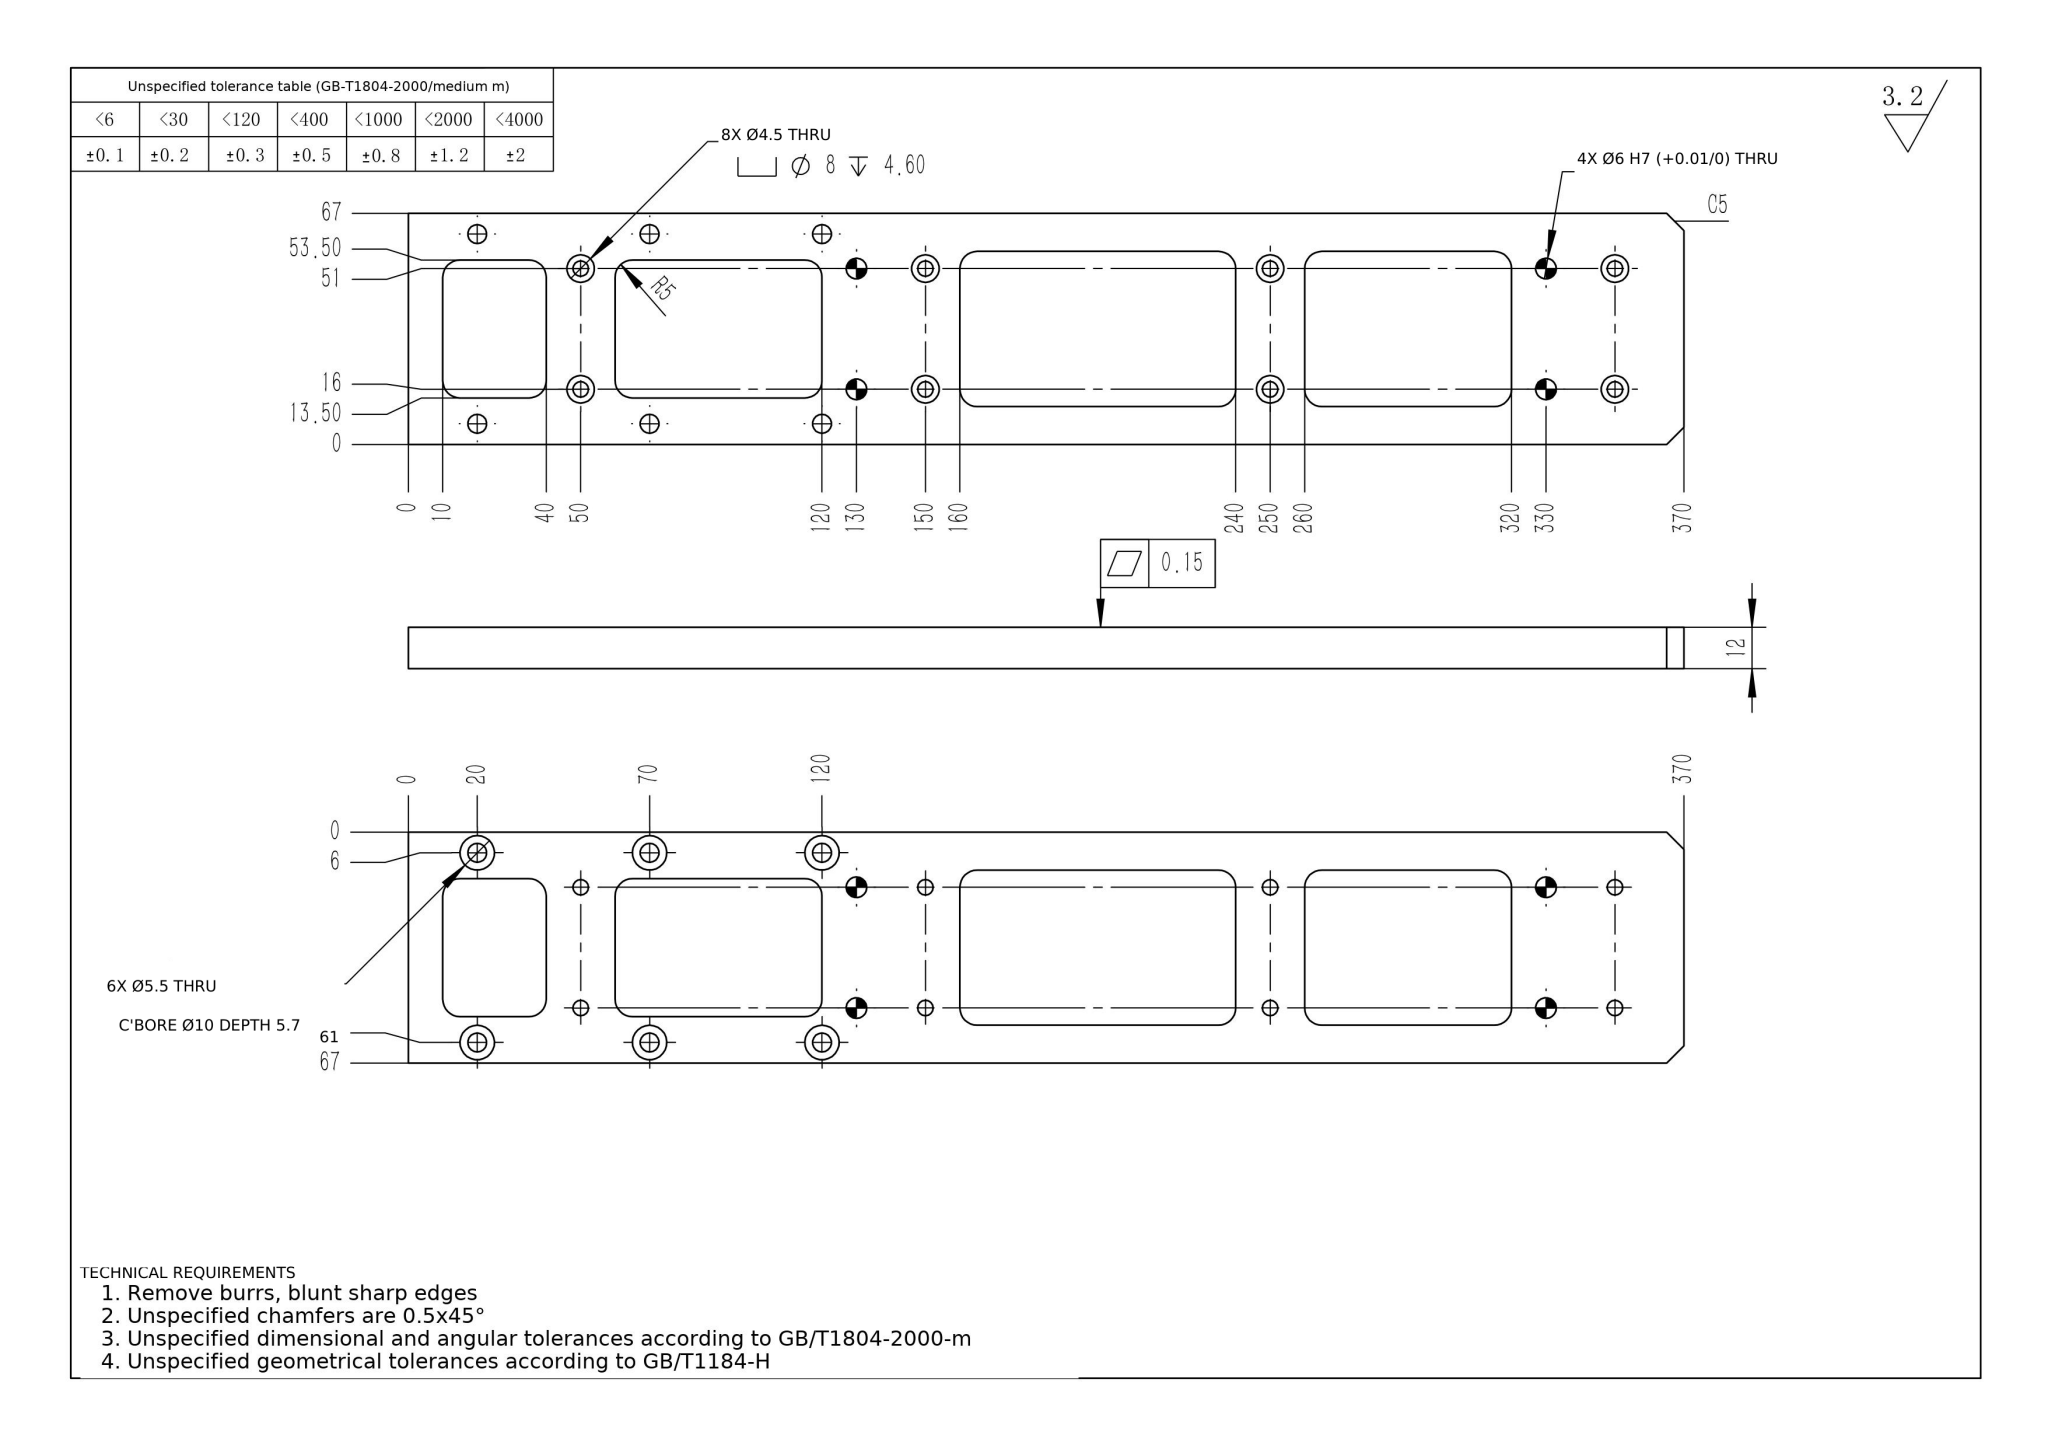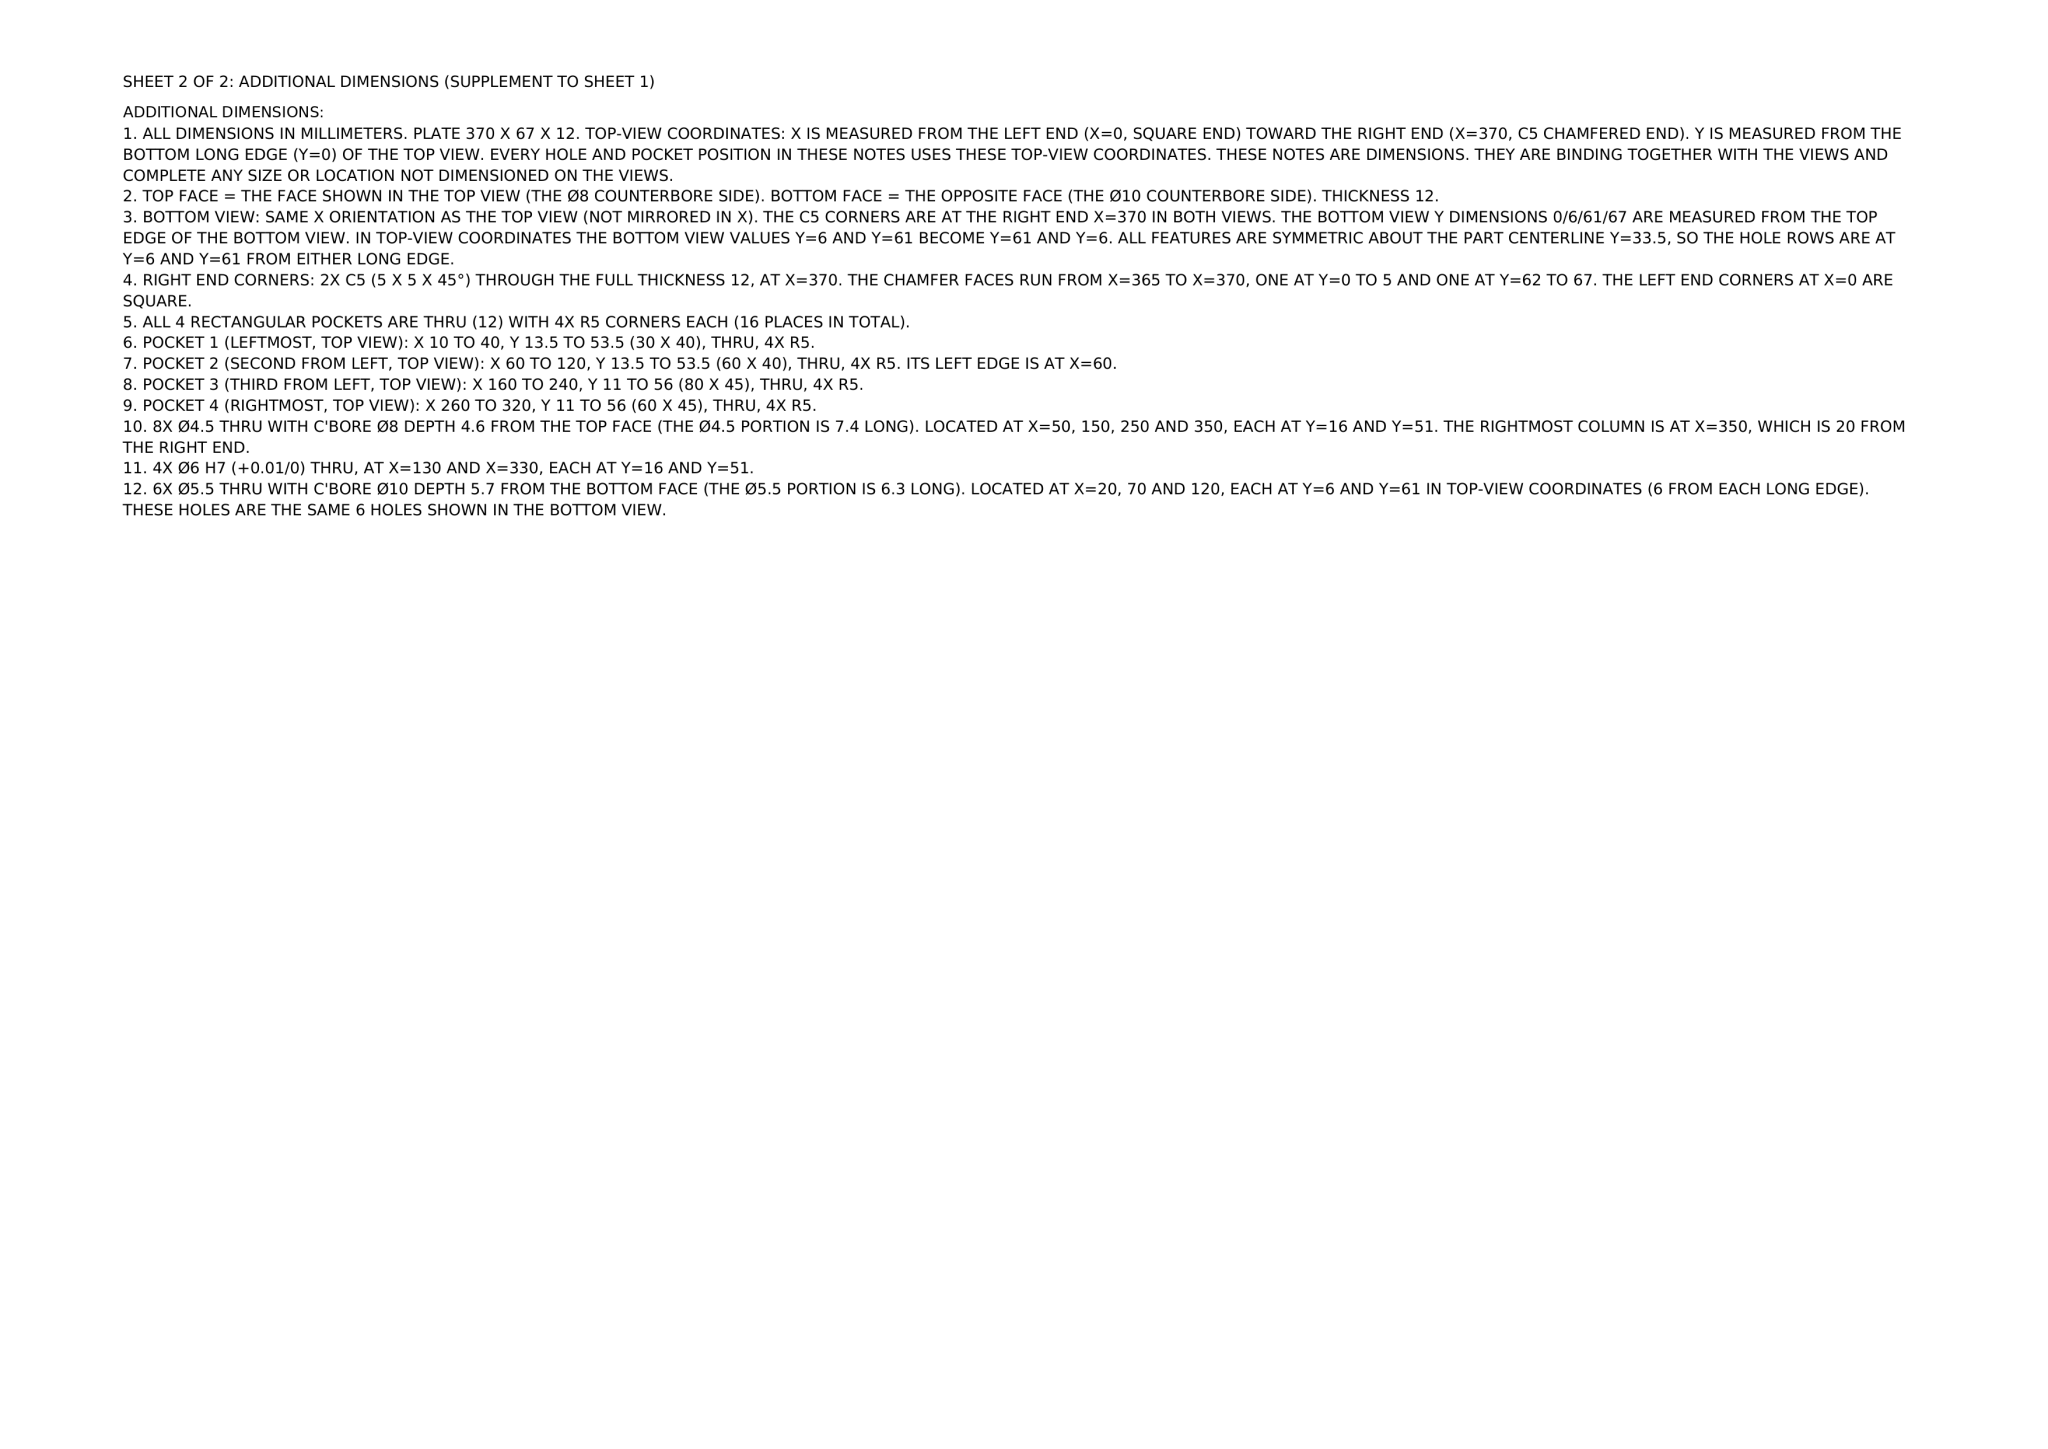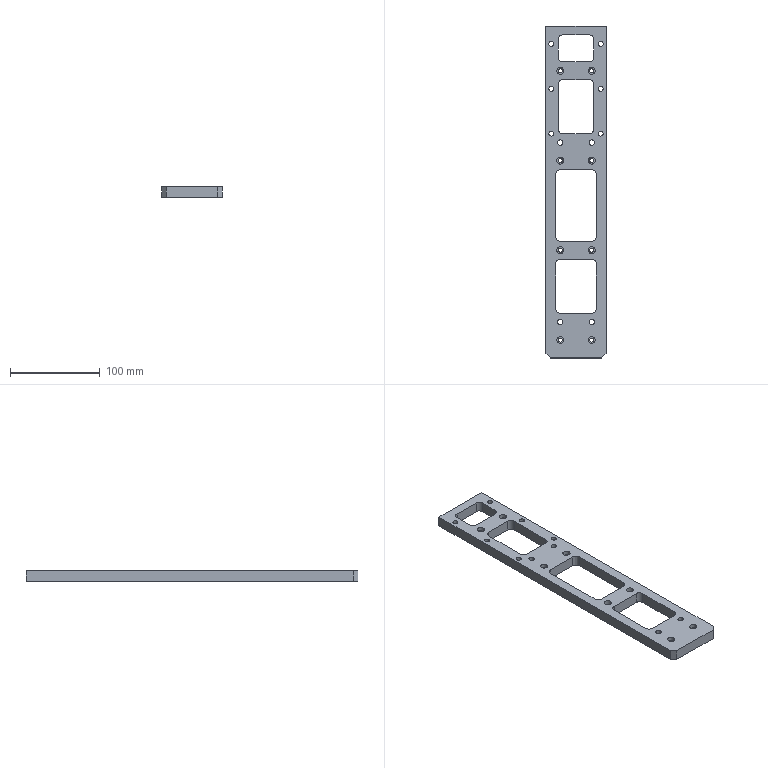Part | NX | mm | 1 solid | 118 faces | box 67 x 370 x 12 mm | volume 171677 mm3 | cylinder 80 | plane 38 | commonest cylinder face diameters 10 x28 8 x16 4.5 x16 5.5 x12 6 x8